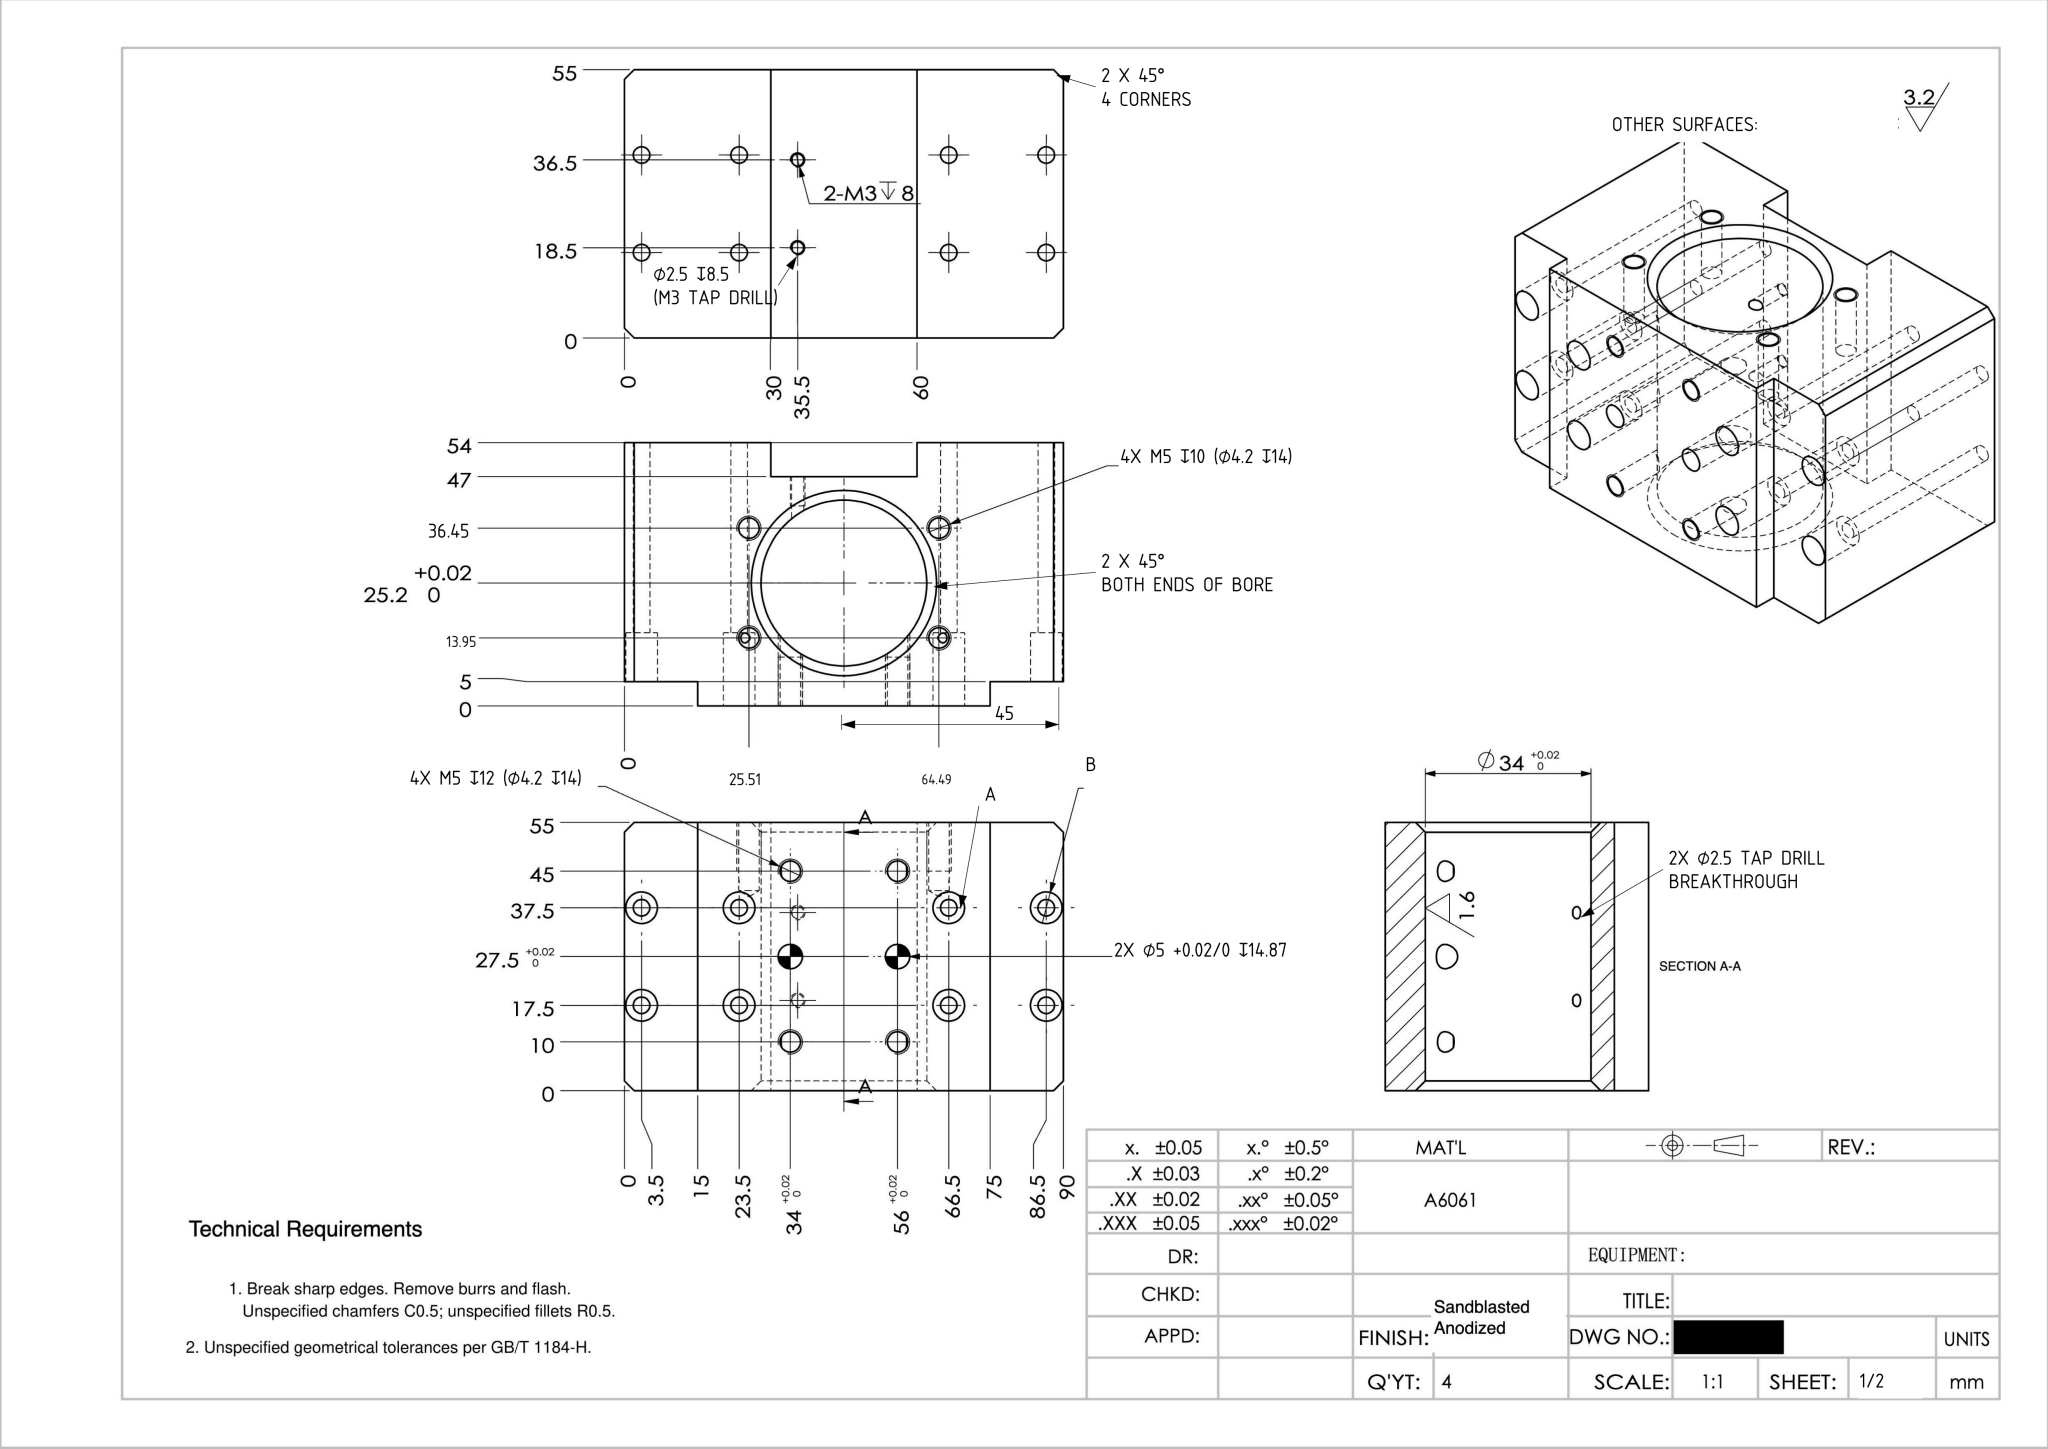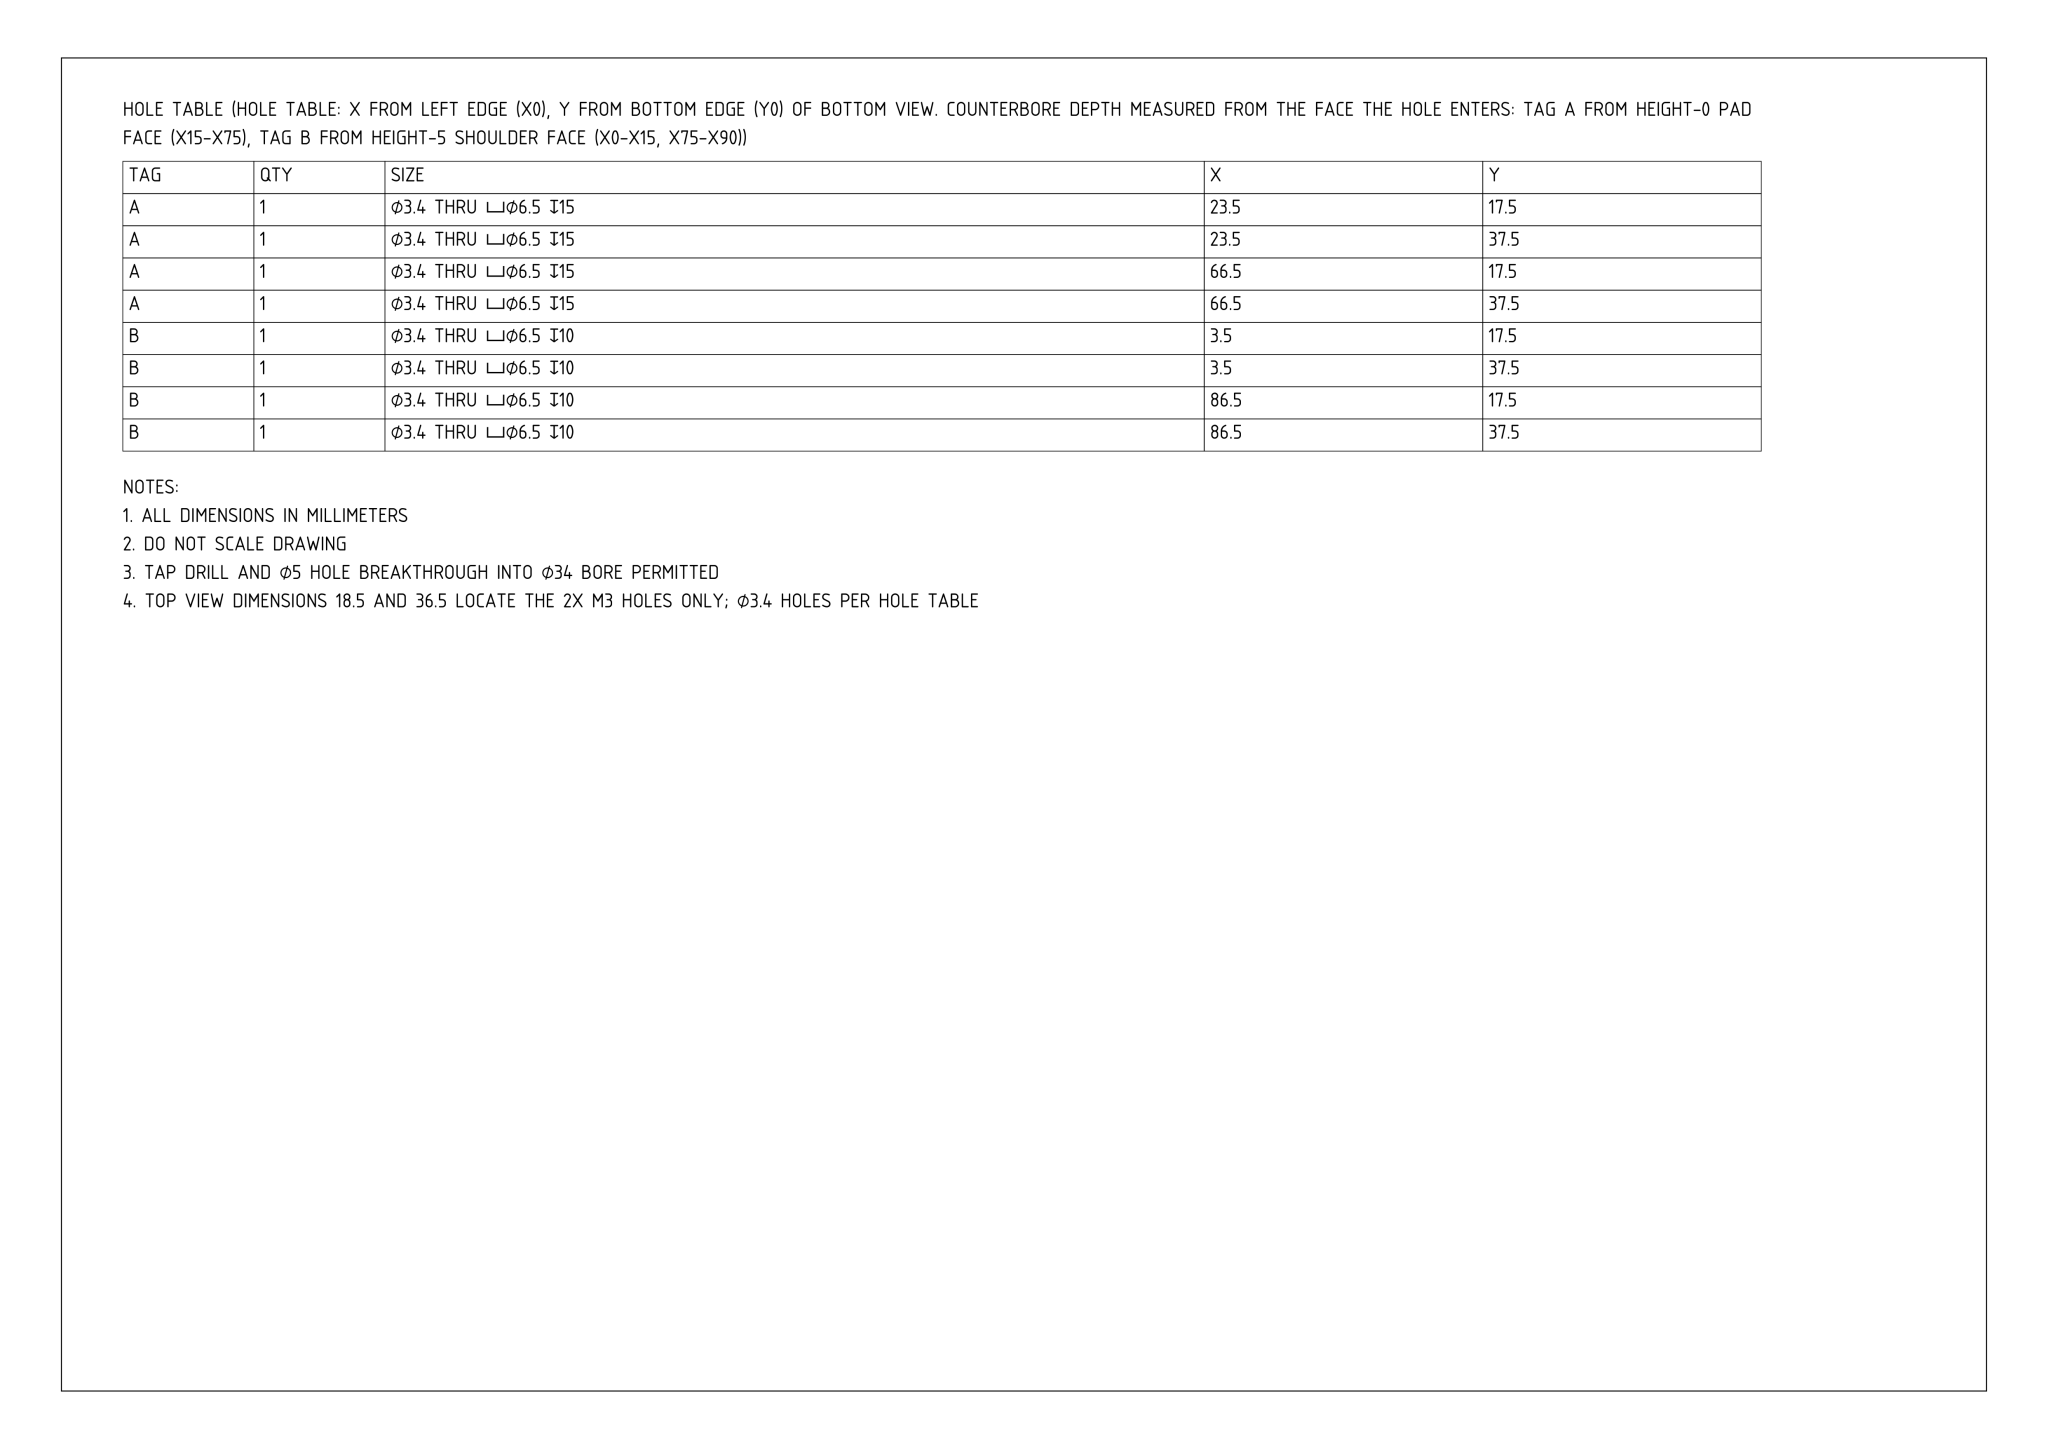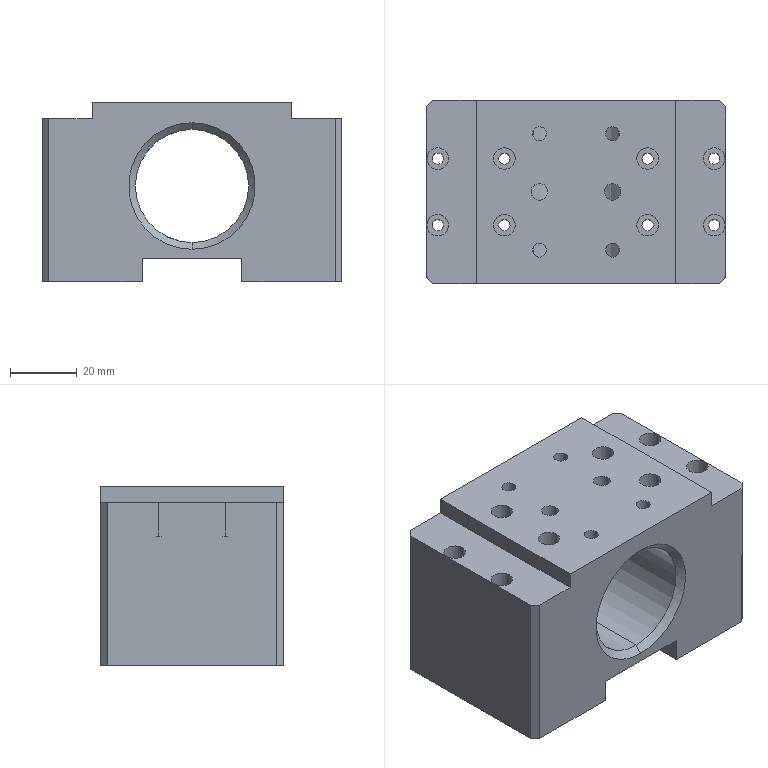Part | NX | mm | 1 solid | 106 faces | box 90 x 55 x 54 mm | volume 188536 mm3 | cylinder 58 | plane 26 | cone 22 | commonest cylinder face diameters 4.2 x16 6.5 x16 3.4 x16 5 x4 2.5 x4 34 x2